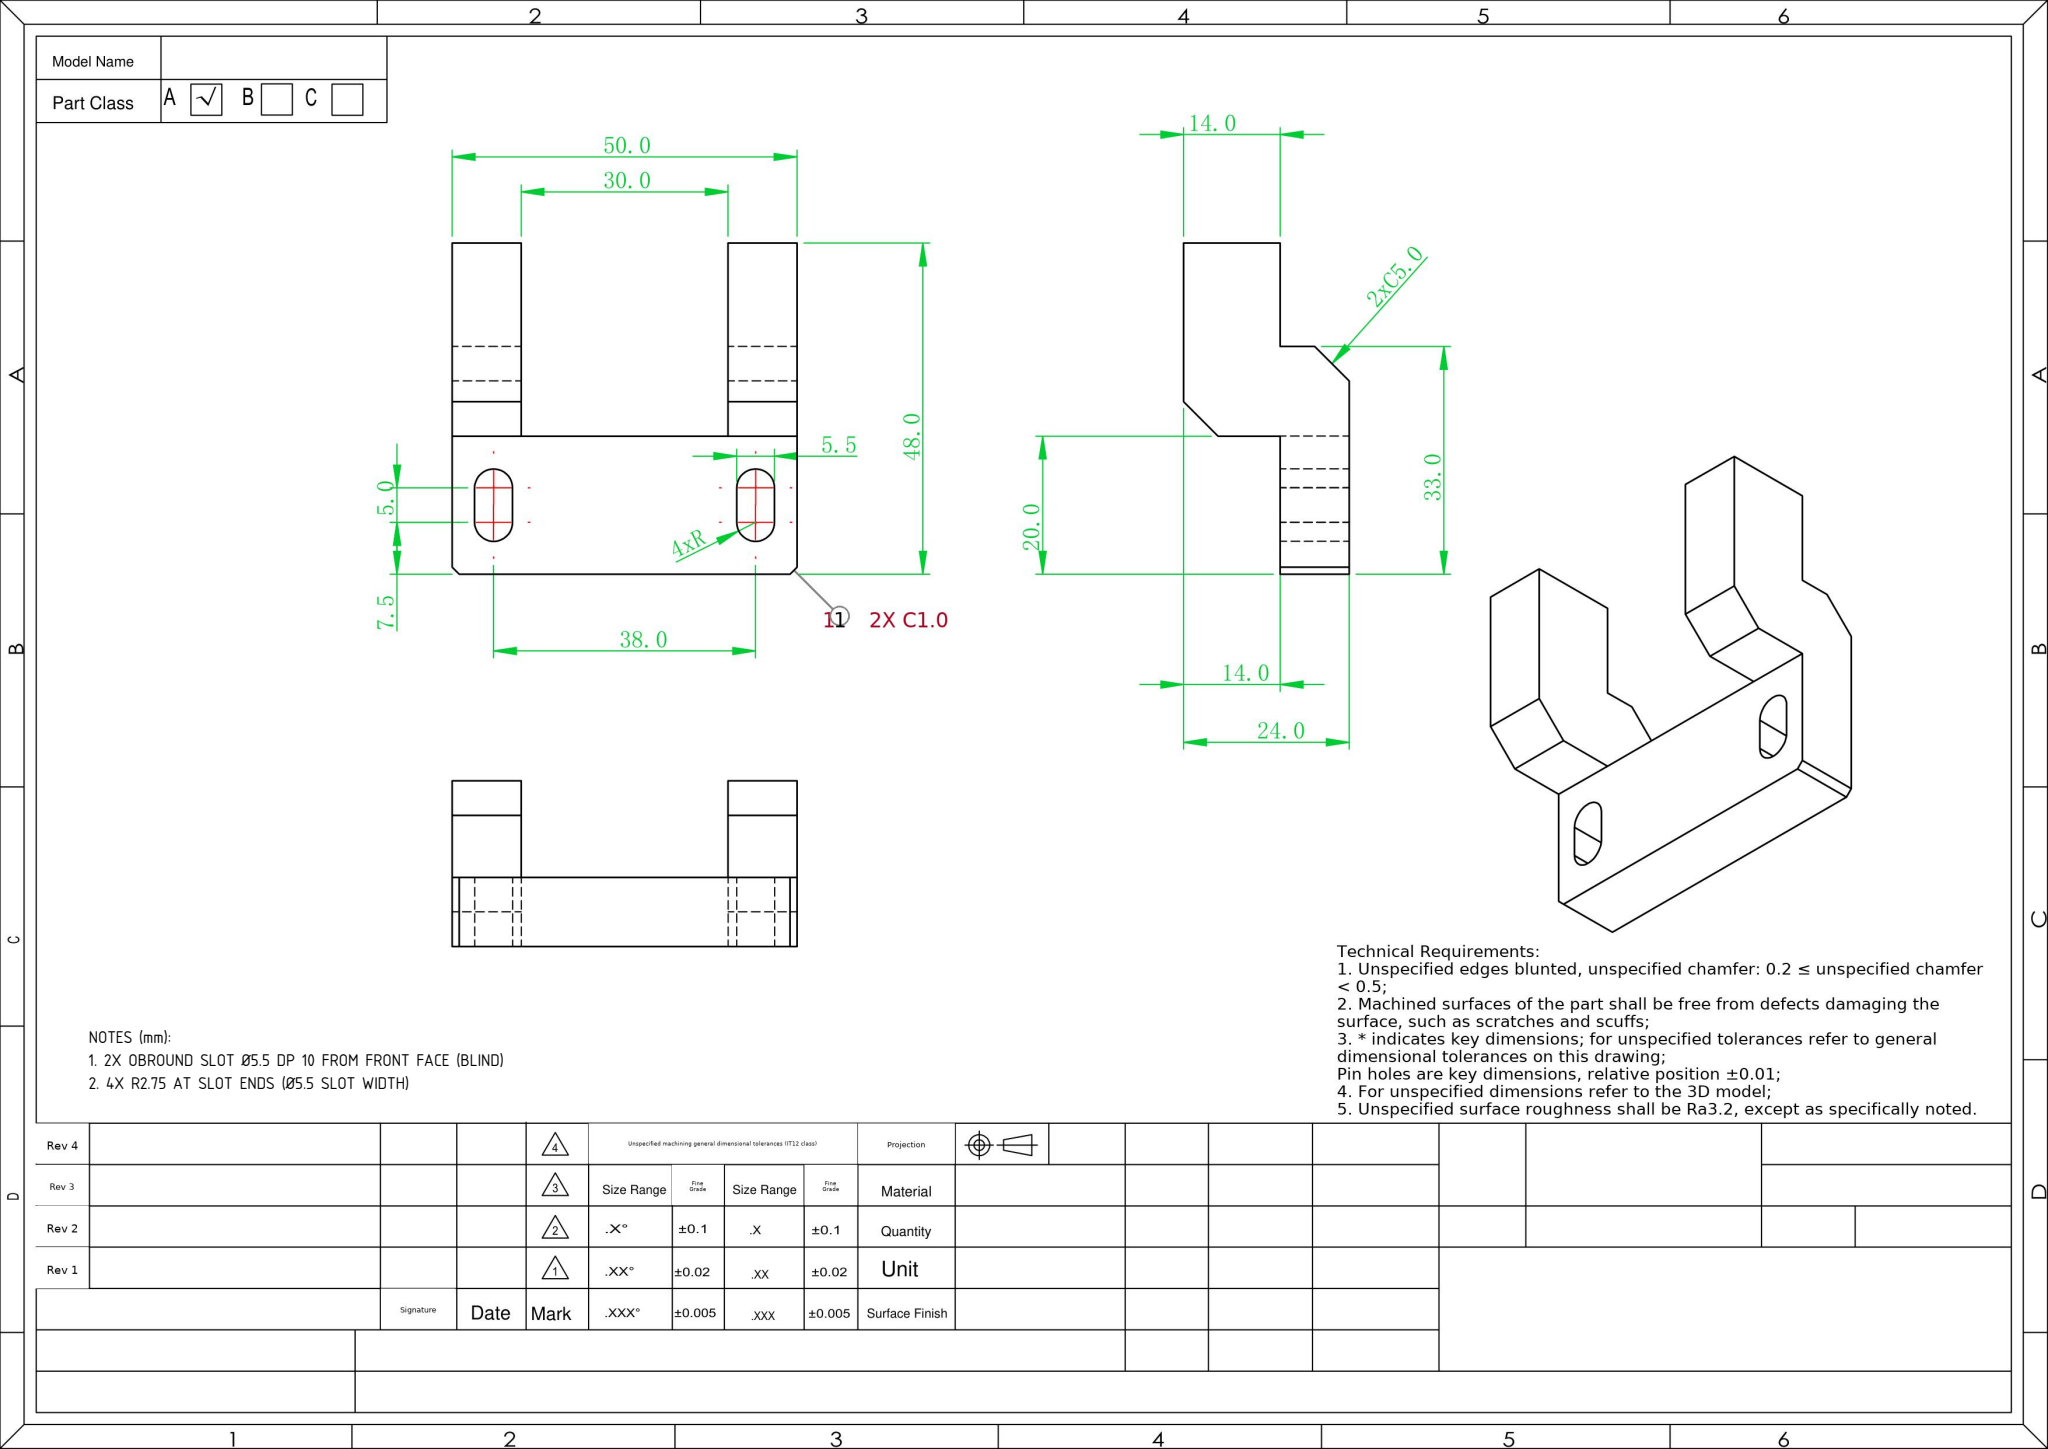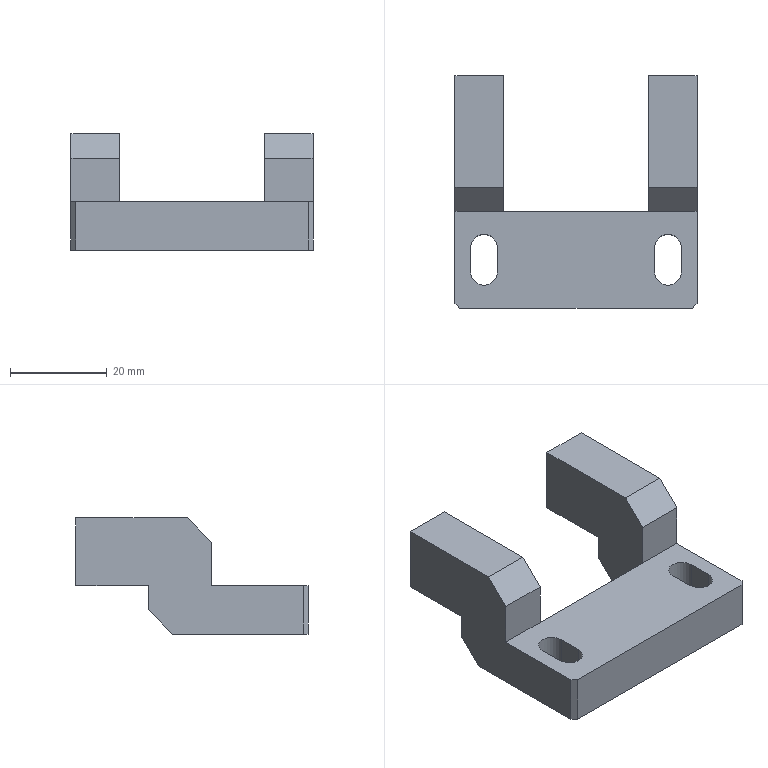Part | SolidWorks | mm | 1 solid | 32 faces | box 50 x 48 x 24 mm | volume 18905 mm3 | plane 28 | cylinder 4 | commonest cylinder face diameters 5.5 x4
Drawing notes:
2X OBROUND SLOT Ø5.5 DP 10 FROM FRONT FACE (BLIND) | from the solid: 4 cylinders Ø5.5, axis z, length 10.0, starting at z=0 (part z-extent 24.0)
4X R2.75 AT SLOT ENDS (Ø5.5 SLOT WIDTH) | from the solid: 4 cylinders dia 5.5 axis z at (6,7.5),(6,12.5),(44,7.5),(44,12.5) -> R2.75 ends
build123d program:
from build123d import *

# Parameters (mm, degrees)
SKETCH1_W           = 50
SKETCH1_H           = 48
BOSS_EXTRUDE1_DEPTH = 24
SKETCH2_W           = 30
SKETCH2_H           = 56
CUT_EXTRUDE1_DEPTH  = 43.154
SKETCH3_W           = 10
SKETCH3_H           = 15
CUT_EXTRUDE2_DEPTH  = 61.432
SKETCH4_W           = 30
SKETCH4_H           = 40
CUT_EXTRUDE4_DEPTH  = 14
SKETCH5_W           = 14
SKETCH5_H           = 20
CUT_EXTRUDE5_DEPTH  = 61.432
CHAMFER2_SIZE       = 5
CUT_EXTRUDE6_DEPTH  = 38.376
CHAMFER3_SIZE       = 1


with BuildPart() as part:
    # Sketch1 → Boss-Extrude1 (new body)
    with BuildSketch(Plane.XY):
        Rectangle(SKETCH1_W, SKETCH1_H)
    extrude(amount=BOSS_EXTRUDE1_DEPTH)

    # Sketch2 → Cut-Extrude1 (cut, through all)
    with BuildSketch(Plane.XY.offset(24)):
        with Locations((0, 24)):
            Rectangle(SKETCH2_W, SKETCH2_H)
    extrude(amount=-CUT_EXTRUDE1_DEPTH, mode=Mode.SUBTRACT)

    # Sketch3 → Cut-Extrude2 (cut, through all)
    with BuildSketch(Plane.ZY.offset(25)):
        with Locations((5, 16.5)):
            Rectangle(SKETCH3_W, SKETCH3_H)
    extrude(amount=-CUT_EXTRUDE2_DEPTH, mode=Mode.SUBTRACT)

    # Sketch4 → Cut-Extrude4 (cut)
    with BuildSketch(Plane.XY.offset(24)):
        with Locations((0, -4)):
            Rectangle(SKETCH4_W, SKETCH4_H)
    extrude(amount=-CUT_EXTRUDE4_DEPTH, mode=Mode.SUBTRACT)

    # Sketch5 → Cut-Extrude5 (cut, through all)
    with BuildSketch(Plane.ZY.offset(25)):
        with Locations((17, -14)):
            Rectangle(SKETCH5_W, SKETCH5_H)
    extrude(amount=-CUT_EXTRUDE5_DEPTH, mode=Mode.SUBTRACT)

    # Chamfer2
    chamfer2_edges = [part.edges().sort_by_distance(p)[0] for p in [
        (20, 9, 0),
        (-20, 9, 0),
        (20, -4, 24),
        (-20, -4, 24),
    ]]
    chamfer(chamfer2_edges, length=CHAMFER2_SIZE)

    # Sketch6 → Cut-Extrude6 (cut, through all)
    with BuildSketch(Plane.XY.offset(10)):
        with BuildLine():
            Line((-16.25, -11.5), (-16.25, -16.5))
            ThreePointArc((-16.25, -16.5), (-19, -19.25), (-21.75, -16.5))
            Line((-21.75, -16.5), (-21.75, -11.5))
            ThreePointArc((-21.75, -11.5), (-19, -8.75), (-16.25, -11.5))
        make_face()
        with BuildLine():
            Line((21.75, -11.5), (21.75, -16.5))
            ThreePointArc((21.75, -16.5), (19, -19.25), (16.25, -16.5))
            Line((16.25, -16.5), (16.25, -11.5))
            ThreePointArc((16.25, -11.5), (19, -8.75), (21.75, -11.5))
        make_face()
    extrude(amount=-CUT_EXTRUDE6_DEPTH, mode=Mode.SUBTRACT)

    # Chamfer3
    chamfer3_edges = [part.edges().sort_by_distance(p)[0] for p in [
        (25, -24, 5),
        (-25, -24, 5),
    ]]
    chamfer(chamfer3_edges, length=CHAMFER3_SIZE)


solid = part.part
STEP:
#1=CARTESIAN_POINT('',(15.,1.,24.));
#2=VERTEX_POINT('',#1);
#3=CARTESIAN_POINT('',(15.,24.,24.));
#4=VERTEX_POINT('',#3);
#5=CARTESIAN_POINT('',(15.,52.,24.));
#6=DIRECTION('',(-0.,1.,0.));
#7=VECTOR('',#6,1000.);
#8=LINE('',#5,#7);
#9=EDGE_CURVE('',#2,#4,#8,.T.);
#10=ORIENTED_EDGE('',*,*,#9,.F.);
#11=CARTESIAN_POINT('',(25.,1.,24.));
#12=VERTEX_POINT('',#11);
#13=CARTESIAN_POINT('',(25.,1.,24.));
#14=DIRECTION('',(1.,0.,0.));
#15=VECTOR('',#14,1000.);
#16=LINE('',#13,#15);
#17=EDGE_CURVE('',#2,#12,#16,.T.);
#18=ORIENTED_EDGE('',*,*,#17,.T.);
#19=CARTESIAN_POINT('',(25.,24.,24.));
#20=VERTEX_POINT('',#19);
#21=CARTESIAN_POINT('',(25.,-24.,24.));
#22=DIRECTION('',(0.,1.,0.));
#23=VECTOR('',#22,1000.);
#24=LINE('',#21,#23);
#25=EDGE_CURVE('',#12,#20,#24,.T.);
#26=ORIENTED_EDGE('',*,*,#25,.T.);
#27=CARTESIAN_POINT('',(25.,24.,24.));
#28=DIRECTION('',(-1.,-0.,0.));
#29=VECTOR('',#28,1000.);
#30=LINE('',#27,#29);
#31=EDGE_CURVE('',#20,#4,#30,.T.);
#32=ORIENTED_EDGE('',*,*,#31,.T.);
#33=EDGE_LOOP('',(#10,#18,#26,#32));
#34=FACE_OUTER_BOUND('',#33,.T.);
#35=CARTESIAN_POINT('',(0.,0.,24.));
#36=DIRECTION('',(0.,0.,1.));
#37=DIRECTION('',(1.,0.,0.));
#38=AXIS2_PLACEMENT_3D('',#35,#36,#37);
#39=PLANE('',#38);
#40=ADVANCED_FACE('',(#34),#39,.T.);
#41=CARTESIAN_POINT('',(15.,-4.,10.));
#42=VERTEX_POINT('',#41);
#43=CARTESIAN_POINT('',(-15.,-4.,10.));
#44=VERTEX_POINT('',#43);
#45=CARTESIAN_POINT('',(-15.,-4.,10.));
#46=DIRECTION('',(-1.,0.,0.));
#47=VECTOR('',#46,1000.);
#48=LINE('',#45,#47);
#49=EDGE_CURVE('',#42,#44,#48,.T.);
#50=ORIENTED_EDGE('',*,*,#49,.F.);
#51=CARTESIAN_POINT('',(15.,-4.,0.));
#52=VERTEX_POINT('',#51);
#53=CARTESIAN_POINT('',(15.,-4.,0.));
#54=DIRECTION('',(0.,0.,1.));
#55=VECTOR('',#54,1000.);
#56=LINE('',#53,#55);
#57=EDGE_CURVE('',#52,#42,#56,.T.);
#58=ORIENTED_EDGE('',*,*,#57,.F.);
#59=CARTESIAN_POINT('',(-15.,-4.,0.));
#60=VERTEX_POINT('',#59);
#61=CARTESIAN_POINT('',(-15.,-4.,0.));
#62=DIRECTION('',(1.,0.,0.));
#63=VECTOR('',#62,1000.);
#64=LINE('',#61,#63);
#65=EDGE_CURVE('',#60,#52,#64,.T.);
#66=ORIENTED_EDGE('',*,*,#65,.F.);
#67=CARTESIAN_POINT('',(-15.,-4.,0.));
#68=DIRECTION('',(0.,0.,1.));
#69=VECTOR('',#68,1000.);
#70=LINE('',#67,#69);
#71=EDGE_CURVE('',#60,#44,#70,.T.);
#72=ORIENTED_EDGE('',*,*,#71,.T.);
#73=EDGE_LOOP('',(#50,#58,#66,#72));
#74=FACE_OUTER_BOUND('',#73,.T.);
#75=CARTESIAN_POINT('',(-15.,-4.,0.));
#76=DIRECTION('',(0.,-1.,0.));
#77=DIRECTION('',(0.,0.,-1.));
#78=AXIS2_PLACEMENT_3D('',#75,#76,#77);
#79=PLANE('',#78);
#80=ADVANCED_FACE('',(#74),#79,.F.);
#81=CARTESIAN_POINT('',(25.,24.,10.));
#82=VERTEX_POINT('',#81);
#83=CARTESIAN_POINT('',(25.,24.,24.));
#84=DIRECTION('',(0.,0.,-1.));
#85=VECTOR('',#84,1000.);
#86=LINE('',#83,#85);
#87=EDGE_CURVE('',#20,#82,#86,.T.);
#88=ORIENTED_EDGE('',*,*,#87,.T.);
#89=CARTESIAN_POINT('',(15.,24.,10.));
#90=VERTEX_POINT('',#89);
#91=CARTESIAN_POINT('',(25.,24.,10.));
#92=DIRECTION('',(-1.,0.,0.));
#93=VECTOR('',#92,1000.);
#94=LINE('',#91,#93);
#95=EDGE_CURVE('',#82,#90,#94,.T.);
#96=ORIENTED_EDGE('',*,*,#95,.T.);
#97=CARTESIAN_POINT('',(15.,24.,24.));
#98=DIRECTION('',(0.,0.,1.));
#99=VECTOR('',#98,1000.);
#100=LINE('',#97,#99);
#101=EDGE_CURVE('',#90,#4,#100,.T.);
#102=ORIENTED_EDGE('',*,*,#101,.T.);
#103=ORIENTED_EDGE('',*,*,#31,.F.);
#104=EDGE_LOOP('',(#88,#96,#102,#103));
#105=FACE_OUTER_BOUND('',#104,.T.);
#106=CARTESIAN_POINT('',(25.,24.,24.));
#107=DIRECTION('',(0.,-1.,0.));
#108=DIRECTION('',(1.,0.,0.));
#109=AXIS2_PLACEMENT_3D('',#106,#107,#108);
#110=PLANE('',#109);
#111=ADVANCED_FACE('',(#105),#110,.F.);
#112=CARTESIAN_POINT('',(-25.,4.,0.));
#113=VERTEX_POINT('',#112);
#114=CARTESIAN_POINT('',(-25.,-23.,0.));
#115=VERTEX_POINT('',#114);
#116=CARTESIAN_POINT('',(-25.,-24.,0.));
#117=DIRECTION('',(0.,-1.,0.));
#118=VECTOR('',#117,1000.);
#119=LINE('',#116,#118);
#120=EDGE_CURVE('',#113,#115,#119,.T.);
#121=ORIENTED_EDGE('',*,*,#120,.T.);
#122=CARTESIAN_POINT('',(-25.,-23.,10.));
#123=VERTEX_POINT('',#122);
#124=CARTESIAN_POINT('',(-25.,-23.,24.));
#125=DIRECTION('',(0.,0.,1.));
#126=VECTOR('',#125,1000.);
#127=LINE('',#124,#126);
#128=EDGE_CURVE('',#115,#123,#127,.T.);
#129=ORIENTED_EDGE('',*,*,#128,.T.);
#130=CARTESIAN_POINT('',(-25.,-4.,10.));
#131=VERTEX_POINT('',#130);
#132=CARTESIAN_POINT('',(-25.,-24.,10.));
#133=DIRECTION('',(0.,-1.,0.));
#134=VECTOR('',#133,1000.);
#135=LINE('',#132,#134);
#136=EDGE_CURVE('',#131,#123,#135,.T.);
#137=ORIENTED_EDGE('',*,*,#136,.F.);
#138=CARTESIAN_POINT('',(-25.,-4.,19.));
#139=VERTEX_POINT('',#138);
#140=CARTESIAN_POINT('',(-25.,-4.,24.));
#141=DIRECTION('',(0.,0.,-1.));
#142=VECTOR('',#141,1000.);
#143=LINE('',#140,#142);
#144=EDGE_CURVE('',#139,#131,#143,.T.);
#145=ORIENTED_EDGE('',*,*,#144,.F.);
#146=CARTESIAN_POINT('',(-25.,1.,24.));
#147=VERTEX_POINT('',#146);
#148=CARTESIAN_POINT('',(-25.,-4.,19.));
#149=DIRECTION('',(0.,0.7071,0.7071));
#150=VECTOR('',#149,1000.);
#151=LINE('',#148,#150);
#152=EDGE_CURVE('',#139,#147,#151,.T.);
#153=ORIENTED_EDGE('',*,*,#152,.T.);
#154=CARTESIAN_POINT('',(-25.,24.,24.));
#155=VERTEX_POINT('',#154);
#156=CARTESIAN_POINT('',(-25.,-24.,24.));
#157=DIRECTION('',(0.,-1.,0.));
#158=VECTOR('',#157,1000.);
#159=LINE('',#156,#158);
#160=EDGE_CURVE('',#155,#147,#159,.T.);
#161=ORIENTED_EDGE('',*,*,#160,.F.);
#162=CARTESIAN_POINT('',(-25.,24.,10.));
#163=VERTEX_POINT('',#162);
#164=CARTESIAN_POINT('',(-25.,24.,24.));
#165=DIRECTION('',(0.,0.,-1.));
#166=VECTOR('',#165,1000.);
#167=LINE('',#164,#166);
#168=EDGE_CURVE('',#155,#163,#167,.T.);
#169=ORIENTED_EDGE('',*,*,#168,.T.);
#170=CARTESIAN_POINT('',(-25.,9.,10.));
#171=VERTEX_POINT('',#170);
#172=CARTESIAN_POINT('',(-25.,24.,10.));
#173=DIRECTION('',(0.,1.,0.));
#174=VECTOR('',#173,1000.);
#175=LINE('',#172,#174);
#176=EDGE_CURVE('',#171,#163,#175,.T.);
#177=ORIENTED_EDGE('',*,*,#176,.F.);
#178=CARTESIAN_POINT('',(-25.,9.,5.));
#179=VERTEX_POINT('',#178);
#180=CARTESIAN_POINT('',(-25.,9.,0.));
#181=DIRECTION('',(0.,0.,1.));
#182=VECTOR('',#181,1000.);
#183=LINE('',#180,#182);
#184=EDGE_CURVE('',#179,#171,#183,.T.);
#185=ORIENTED_EDGE('',*,*,#184,.F.);
#186=CARTESIAN_POINT('',(-25.,9.,5.));
#187=DIRECTION('',(0.,-0.7071,-0.7071));
#188=VECTOR('',#187,1000.);
#189=LINE('',#186,#188);
#190=EDGE_CURVE('',#179,#113,#189,.T.);
#191=ORIENTED_EDGE('',*,*,#190,.T.);
#192=EDGE_LOOP('',(#121,#129,#137,#145,#153,#161,#169,#177,#185,#191));
#193=FACE_OUTER_BOUND('',#192,.T.);
#194=CARTESIAN_POINT('',(-25.,-24.,24.));
#195=DIRECTION('',(1.,0.,0.));
#196=DIRECTION('',(0.,0.,-1.));
#197=AXIS2_PLACEMENT_3D('',#194,#195,#196);
#198=PLANE('',#197);
#199=ADVANCED_FACE('',(#193),#198,.F.);
#200=CARTESIAN_POINT('',(-24.,-24.,0.));
#201=VERTEX_POINT('',#200);
#202=CARTESIAN_POINT('',(24.,-24.,0.));
#203=VERTEX_POINT('',#202);
#204=CARTESIAN_POINT('',(25.,-24.,0.));
#205=DIRECTION('',(1.,0.,0.));
#206=VECTOR('',#205,1000.);
#207=LINE('',#204,#206);
#208=EDGE_CURVE('',#201,#203,#207,.T.);
#209=ORIENTED_EDGE('',*,*,#208,.T.);
#210=CARTESIAN_POINT('',(24.,-24.,10.));
#211=VERTEX_POINT('',#210);
#212=CARTESIAN_POINT('',(24.,-24.,24.));
#213=DIRECTION('',(0.,0.,1.));
#214=VECTOR('',#213,1000.);
#215=LINE('',#212,#214);
#216=EDGE_CURVE('',#203,#211,#215,.T.);
#217=ORIENTED_EDGE('',*,*,#216,.T.);
#218=CARTESIAN_POINT('',(-24.,-24.,10.));
#219=VERTEX_POINT('',#218);
#220=CARTESIAN_POINT('',(-15.,-24.,10.));
#221=DIRECTION('',(1.,0.,0.));
#222=VECTOR('',#221,1000.);
#223=LINE('',#220,#222);
#224=EDGE_CURVE('',#219,#211,#223,.T.);
#225=ORIENTED_EDGE('',*,*,#224,.F.);
#226=CARTESIAN_POINT('',(-24.,-24.,24.));
#227=DIRECTION('',(0.,0.,-1.));
#228=VECTOR('',#227,1000.);
#229=LINE('',#226,#228);
#230=EDGE_CURVE('',#219,#201,#229,.T.);
#231=ORIENTED_EDGE('',*,*,#230,.T.);
#232=EDGE_LOOP('',(#209,#217,#225,#231));
#233=FACE_OUTER_BOUND('',#232,.T.);
#234=CARTESIAN_POINT('',(25.,-24.,24.));
#235=DIRECTION('',(-0.,1.,0.));
#236=DIRECTION('',(-1.,-0.,0.));
#237=AXIS2_PLACEMENT_3D('',#234,#235,#236);
#238=PLANE('',#237);
#239=ADVANCED_FACE('',(#233),#238,.F.);
#240=CARTESIAN_POINT('',(25.,-4.,10.));
#241=VERTEX_POINT('',#240);
#242=CARTESIAN_POINT('',(25.,-23.,10.));
#243=VERTEX_POINT('',#242);
#244=CARTESIAN_POINT('',(25.,-24.,10.));
#245=DIRECTION('',(0.,-1.,0.));
#246=VECTOR('',#245,1000.);
#247=LINE('',#244,#246);
#248=EDGE_CURVE('',#241,#243,#247,.T.);
#249=ORIENTED_EDGE('',*,*,#248,.T.);
#250=CARTESIAN_POINT('',(25.,-23.,0.));
#251=VERTEX_POINT('',#250);
#252=CARTESIAN_POINT('',(25.,-23.,24.));
#253=DIRECTION('',(0.,0.,-1.));
#254=VECTOR('',#253,1000.);
#255=LINE('',#252,#254);
#256=EDGE_CURVE('',#243,#251,#255,.T.);
#257=ORIENTED_EDGE('',*,*,#256,.T.);
#258=CARTESIAN_POINT('',(25.,4.,0.));
#259=VERTEX_POINT('',#258);
#260=CARTESIAN_POINT('',(25.,-24.,0.));
#261=DIRECTION('',(0.,1.,0.));
#262=VECTOR('',#261,1000.);
#263=LINE('',#260,#262);
#264=EDGE_CURVE('',#251,#259,#263,.T.);
#265=ORIENTED_EDGE('',*,*,#264,.T.);
#266=CARTESIAN_POINT('',(25.,9.,5.));
#267=VERTEX_POINT('',#266);
#268=CARTESIAN_POINT('',(25.,9.,5.));
#269=DIRECTION('',(0.,0.7071,0.7071));
#270=VECTOR('',#269,1000.);
#271=LINE('',#268,#270);
#272=EDGE_CURVE('',#259,#267,#271,.T.);
#273=ORIENTED_EDGE('',*,*,#272,.T.);
#274=CARTESIAN_POINT('',(25.,9.,10.));
#275=VERTEX_POINT('',#274);
#276=CARTESIAN_POINT('',(25.,9.,0.));
#277=DIRECTION('',(0.,0.,1.));
#278=VECTOR('',#277,1000.);
#279=LINE('',#276,#278);
#280=EDGE_CURVE('',#267,#275,#279,.T.);
#281=ORIENTED_EDGE('',*,*,#280,.T.);
#282=CARTESIAN_POINT('',(25.,24.,10.));
#283=DIRECTION('',(0.,1.,0.));
#284=VECTOR('',#283,1000.);
#285=LINE('',#282,#284);
#286=EDGE_CURVE('',#275,#82,#285,.T.);
#287=ORIENTED_EDGE('',*,*,#286,.T.);
#288=ORIENTED_EDGE('',*,*,#87,.F.);
#289=ORIENTED_EDGE('',*,*,#25,.F.);
#290=CARTESIAN_POINT('',(25.,-4.,19.));
#291=VERTEX_POINT('',#290);
#292=CARTESIAN_POINT('',(25.,-4.,19.));
#293=DIRECTION('',(0.,-0.7071,-0.7071));
#294=VECTOR('',#293,1000.);
#295=LINE('',#292,#294);
#296=EDGE_CURVE('',#12,#291,#295,.T.);
#297=ORIENTED_EDGE('',*,*,#296,.T.);
#298=CARTESIAN_POINT('',(25.,-4.,24.));
#299=DIRECTION('',(0.,0.,-1.));
#300=VECTOR('',#299,1000.);
#301=LINE('',#298,#300);
#302=EDGE_CURVE('',#291,#241,#301,.T.);
#303=ORIENTED_EDGE('',*,*,#302,.T.);
#304=EDGE_LOOP('',(#249,#257,#265,#273,#281,#287,#288,#289,#297,#303));
#305=FACE_OUTER_BOUND('',#304,.T.);
#306=CARTESIAN_POINT('',(25.,-24.,24.));
#307=DIRECTION('',(-1.,0.,0.));
#308=DIRECTION('',(0.,0.,1.));
#309=AXIS2_PLACEMENT_3D('',#306,#307,#308);
#310=PLANE('',#309);
#311=ADVANCED_FACE('',(#305),#310,.F.);
#312=CARTESIAN_POINT('',(-15.,24.,24.));
#313=VERTEX_POINT('',#312);
#314=CARTESIAN_POINT('',(-15.,24.,10.));
#315=VERTEX_POINT('',#314);
#316=CARTESIAN_POINT('',(-15.,24.,24.));
#317=DIRECTION('',(0.,0.,-1.));
#318=VECTOR('',#317,1000.);
#319=LINE('',#316,#318);
#320=EDGE_CURVE('',#313,#315,#319,.T.);
#321=ORIENTED_EDGE('',*,*,#320,.T.);
#322=CARTESIAN_POINT('',(25.,24.,10.));
#323=DIRECTION('',(-1.,0.,0.));
#324=VECTOR('',#323,1000.);
#325=LINE('',#322,#324);
#326=EDGE_CURVE('',#315,#163,#325,.T.);
#327=ORIENTED_EDGE('',*,*,#326,.T.);
#328=ORIENTED_EDGE('',*,*,#168,.F.);
#329=CARTESIAN_POINT('',(25.,24.,24.));
#330=DIRECTION('',(-1.,-0.,0.));
#331=VECTOR('',#330,1000.);
#332=LINE('',#329,#331);
#333=EDGE_CURVE('',#313,#155,#332,.T.);
#334=ORIENTED_EDGE('',*,*,#333,.F.);
#335=EDGE_LOOP('',(#321,#327,#328,#334));
#336=FACE_OUTER_BOUND('',#335,.T.);
#337=CARTESIAN_POINT('',(25.,24.,24.));
#338=DIRECTION('',(0.,-1.,0.));
#339=DIRECTION('',(1.,0.,0.));
#340=AXIS2_PLACEMENT_3D('',#337,#338,#339);
#341=PLANE('',#340);
#342=ADVANCED_FACE('',(#336),#341,.F.);
#343=ORIENTED_EDGE('',*,*,#160,.T.);
#344=CARTESIAN_POINT('',(-15.,1.,24.));
#345=VERTEX_POINT('',#344);
#346=CARTESIAN_POINT('',(-15.,1.,24.));
#347=DIRECTION('',(1.,0.,0.));
#348=VECTOR('',#347,1000.);
#349=LINE('',#346,#348);
#350=EDGE_CURVE('',#147,#345,#349,.T.);
#351=ORIENTED_EDGE('',*,*,#350,.T.);
#352=CARTESIAN_POINT('',(-15.,52.,24.));
#353=DIRECTION('',(0.,-1.,0.));
#354=VECTOR('',#353,1000.);
#355=LINE('',#352,#354);
#356=EDGE_CURVE('',#313,#345,#355,.T.);
#357=ORIENTED_EDGE('',*,*,#356,.F.);
#358=ORIENTED_EDGE('',*,*,#333,.T.);
#359=EDGE_LOOP('',(#343,#351,#357,#358));
#360=FACE_OUTER_BOUND('',#359,.T.);
#361=CARTESIAN_POINT('',(0.,0.,24.));
#362=DIRECTION('',(0.,0.,1.));
#363=DIRECTION('',(1.,0.,0.));
#364=AXIS2_PLACEMENT_3D('',#361,#362,#363);
#365=PLANE('',#364);
#366=ADVANCED_FACE('',(#360),#365,.T.);
#367=CARTESIAN_POINT('',(-16.25,-16.5,0.));
#368=VERTEX_POINT('',#367);
#369=CARTESIAN_POINT('',(-16.25,-11.5,0.));
#370=VERTEX_POINT('',#369);
#371=CARTESIAN_POINT('',(-16.25,-11.5,0.));
#372=DIRECTION('',(0.,1.,0.));
#373=VECTOR('',#372,1000.);
#374=LINE('',#371,#373);
#375=EDGE_CURVE('',#368,#370,#374,.T.);
#376=ORIENTED_EDGE('',*,*,#375,.T.);
#377=CARTESIAN_POINT('',(-21.75,-11.5,0.));
#378=VERTEX_POINT('',#377);
#379=CARTESIAN_POINT('',(-19.,-11.5,0.));
#380=DIRECTION('',(0.,0.,1.));
#381=DIRECTION('',(1.,0.,0.));
#382=AXIS2_PLACEMENT_3D('',#379,#380,#381);
#383=CIRCLE('',#382,2.75);
#384=EDGE_CURVE('',#370,#378,#383,.T.);
#385=ORIENTED_EDGE('',*,*,#384,.T.);
#386=CARTESIAN_POINT('',(-21.75,-16.5,0.));
#387=VERTEX_POINT('',#386);
#388=CARTESIAN_POINT('',(-21.75,-11.5,0.));
#389=DIRECTION('',(0.,-1.,0.));
#390=VECTOR('',#389,1000.);
#391=LINE('',#388,#390);
#392=EDGE_CURVE('',#378,#387,#391,.T.);
#393=ORIENTED_EDGE('',*,*,#392,.T.);
#394=CARTESIAN_POINT('',(-19.,-16.5,0.));
#395=DIRECTION('',(0.,0.,1.));
#396=DIRECTION('',(1.,0.,0.));
#397=AXIS2_PLACEMENT_3D('',#394,#395,#396);
#398=CIRCLE('',#397,2.75);
#399=EDGE_CURVE('',#387,#368,#398,.T.);
#400=ORIENTED_EDGE('',*,*,#399,.T.);
#401=EDGE_LOOP('',(#376,#385,#393,#400));
#402=FACE_BOUND('',#401,.T.);
#403=CARTESIAN_POINT('',(21.75,-16.5,0.));
#404=VERTEX_POINT('',#403);
#405=CARTESIAN_POINT('',(21.75,-11.5,0.));
#406=VERTEX_POINT('',#405);
#407=CARTESIAN_POINT('',(21.75,-11.5,0.));
#408=DIRECTION('',(0.,1.,0.));
#409=VECTOR('',#408,1000.);
#410=LINE('',#407,#409);
#411=EDGE_CURVE('',#404,#406,#410,.T.);
#412=ORIENTED_EDGE('',*,*,#411,.T.);
#413=CARTESIAN_POINT('',(16.25,-11.5,0.));
#414=VERTEX_POINT('',#413);
#415=CARTESIAN_POINT('',(19.,-11.5,0.));
#416=DIRECTION('',(0.,0.,1.));
#417=DIRECTION('',(1.,0.,0.));
#418=AXIS2_PLACEMENT_3D('',#415,#416,#417);
#419=CIRCLE('',#418,2.75);
#420=EDGE_CURVE('',#406,#414,#419,.T.);
#421=ORIENTED_EDGE('',*,*,#420,.T.);
#422=CARTESIAN_POINT('',(16.25,-16.5,0.));
#423=VERTEX_POINT('',#422);
#424=CARTESIAN_POINT('',(16.25,-11.5,0.));
#425=DIRECTION('',(0.,-1.,0.));
#426=VECTOR('',#425,1000.);
#427=LINE('',#424,#426);
#428=EDGE_CURVE('',#414,#423,#427,.T.);
#429=ORIENTED_EDGE('',*,*,#428,.T.);
#430=CARTESIAN_POINT('',(19.,-16.5,0.));
#431=DIRECTION('',(0.,0.,1.));
#432=DIRECTION('',(1.,0.,0.));
#433=AXIS2_PLACEMENT_3D('',#430,#431,#432);
#434=CIRCLE('',#433,2.75);
#435=EDGE_CURVE('',#423,#404,#434,.T.);
#436=ORIENTED_EDGE('',*,*,#435,.T.);
#437=EDGE_LOOP('',(#412,#421,#429,#436));
#438=FACE_BOUND('',#437,.T.);
#439=ORIENTED_EDGE('',*,*,#264,.F.);
#440=CARTESIAN_POINT('',(25.,-23.,0.));
#441=DIRECTION('',(-0.7071,-0.7071,0.));
#442=VECTOR('',#441,1000.);
#443=LINE('',#440,#442);
#444=EDGE_CURVE('',#251,#203,#443,.T.);
#445=ORIENTED_EDGE('',*,*,#444,.T.);
#446=ORIENTED_EDGE('',*,*,#208,.F.);
#447=CARTESIAN_POINT('',(-24.,-24.,0.));
#448=DIRECTION('',(-0.7071,0.7071,0.));
#449=VECTOR('',#448,1000.);
#450=LINE('',#447,#449);
#451=EDGE_CURVE('',#201,#115,#450,.T.);
#452=ORIENTED_EDGE('',*,*,#451,.T.);
#453=ORIENTED_EDGE('',*,*,#120,.F.);
#454=CARTESIAN_POINT('',(-15.,4.,0.));
#455=VERTEX_POINT('',#454);
#456=CARTESIAN_POINT('',(0.,4.,0.));
#457=DIRECTION('',(1.,0.,0.));
#458=VECTOR('',#457,1000.);
#459=LINE('',#456,#458);
#460=EDGE_CURVE('',#113,#455,#459,.T.);
#461=ORIENTED_EDGE('',*,*,#460,.T.);
#462=CARTESIAN_POINT('',(-15.,-0.,0.));
#463=DIRECTION('',(0.,-1.,0.));
#464=VECTOR('',#463,1000.);
#465=LINE('',#462,#464);
#466=EDGE_CURVE('',#455,#60,#465,.T.);
#467=ORIENTED_EDGE('',*,*,#466,.T.);
#468=ORIENTED_EDGE('',*,*,#65,.T.);
#469=CARTESIAN_POINT('',(15.,4.,0.));
#470=VERTEX_POINT('',#469);
#471=CARTESIAN_POINT('',(15.,52.,0.));
#472=DIRECTION('',(-0.,1.,0.));
#473=VECTOR('',#472,1000.);
#474=LINE('',#471,#473);
#475=EDGE_CURVE('',#52,#470,#474,.T.);
#476=ORIENTED_EDGE('',*,*,#475,.T.);
#477=CARTESIAN_POINT('',(0.,4.,0.));
#478=DIRECTION('',(1.,0.,0.));
#479=VECTOR('',#478,1000.);
#480=LINE('',#477,#479);
#481=EDGE_CURVE('',#470,#259,#480,.T.);
#482=ORIENTED_EDGE('',*,*,#481,.T.);
#483=EDGE_LOOP('',(#439,#445,#446,#452,#453,#461,#467,#468,#476,#482));
#484=FACE_OUTER_BOUND('',#483,.T.);
#485=CARTESIAN_POINT('',(0.,0.,0.));
#486=DIRECTION('',(0.,0.,1.));
#487=DIRECTION('',(1.,0.,0.));
#488=AXIS2_PLACEMENT_3D('',#485,#486,#487);
#489=PLANE('',#488);
#490=ADVANCED_FACE('',(#402,#438,#484),#489,.F.);
#491=CARTESIAN_POINT('',(15.,-4.,19.));
#492=VERTEX_POINT('',#491);
#493=CARTESIAN_POINT('',(15.,-4.,0.));
#494=DIRECTION('',(0.,0.,1.));
#495=VECTOR('',#494,1000.);
#496=LINE('',#493,#495);
#497=EDGE_CURVE('',#42,#492,#496,.T.);
#498=ORIENTED_EDGE('',*,*,#497,.T.);
#499=CARTESIAN_POINT('',(15.,-4.,19.));
#500=DIRECTION('',(-0.,0.7071,0.7071));
#501=VECTOR('',#500,1000.);
#502=LINE('',#499,#501);
#503=EDGE_CURVE('',#492,#2,#502,.T.);
#504=ORIENTED_EDGE('',*,*,#503,.T.);
#505=ORIENTED_EDGE('',*,*,#9,.T.);
#506=ORIENTED_EDGE('',*,*,#101,.F.);
#507=CARTESIAN_POINT('',(15.,9.,10.));
#508=VERTEX_POINT('',#507);
#509=CARTESIAN_POINT('',(15.,52.,10.));
#510=DIRECTION('',(0.,-1.,0.));
#511=VECTOR('',#510,1000.);
#512=LINE('',#509,#511);
#513=EDGE_CURVE('',#90,#508,#512,.T.);
#514=ORIENTED_EDGE('',*,*,#513,.T.);
#515=CARTESIAN_POINT('',(15.,9.,5.));
#516=VERTEX_POINT('',#515);
#517=CARTESIAN_POINT('',(15.,9.,0.));
#518=DIRECTION('',(0.,0.,-1.));
#519=VECTOR('',#518,1000.);
#520=LINE('',#517,#519);
#521=EDGE_CURVE('',#508,#516,#520,.T.);
#522=ORIENTED_EDGE('',*,*,#521,.T.);
#523=CARTESIAN_POINT('',(15.,9.,5.));
#524=DIRECTION('',(0.,-0.7071,-0.7071));
#525=VECTOR('',#524,1000.);
#526=LINE('',#523,#525);
#527=EDGE_CURVE('',#516,#470,#526,.T.);
#528=ORIENTED_EDGE('',*,*,#527,.T.);
#529=ORIENTED_EDGE('',*,*,#475,.F.);
#530=ORIENTED_EDGE('',*,*,#57,.T.);
#531=EDGE_LOOP('',(#498,#504,#505,#506,#514,#522,#528,#529,#530));
#532=FACE_OUTER_BOUND('',#531,.T.);
#533=CARTESIAN_POINT('',(15.,52.,0.));
#534=DIRECTION('',(1.,0.,0.));
#535=DIRECTION('',(-0.,1.,0.));
#536=AXIS2_PLACEMENT_3D('',#533,#534,#535);
#537=PLANE('',#536);
#538=ADVANCED_FACE('',(#532),#537,.F.);
#539=ORIENTED_EDGE('',*,*,#356,.T.);
#540=CARTESIAN_POINT('',(-15.,-4.,19.));
#541=VERTEX_POINT('',#540);
#542=CARTESIAN_POINT('',(-15.,-4.,19.));
#543=DIRECTION('',(0.,-0.7071,-0.7071));
#544=VECTOR('',#543,1000.);
#545=LINE('',#542,#544);
#546=EDGE_CURVE('',#345,#541,#545,.T.);
#547=ORIENTED_EDGE('',*,*,#546,.T.);
#548=CARTESIAN_POINT('',(-15.,-4.,0.));
#549=DIRECTION('',(0.,0.,-1.));
#550=VECTOR('',#549,1000.);
#551=LINE('',#548,#550);
#552=EDGE_CURVE('',#541,#44,#551,.T.);
#553=ORIENTED_EDGE('',*,*,#552,.T.);
#554=ORIENTED_EDGE('',*,*,#71,.F.);
#555=ORIENTED_EDGE('',*,*,#466,.F.);
#556=CARTESIAN_POINT('',(-15.,9.,5.));
#557=VERTEX_POINT('',#556);
#558=CARTESIAN_POINT('',(-15.,9.,5.));
#559=DIRECTION('',(-0.,0.7071,0.7071));
#560=VECTOR('',#559,1000.);
#561=LINE('',#558,#560);
#562=EDGE_CURVE('',#455,#557,#561,.T.);
#563=ORIENTED_EDGE('',*,*,#562,.T.);
#564=CARTESIAN_POINT('',(-15.,9.,10.));
#565=VERTEX_POINT('',#564);
#566=CARTESIAN_POINT('',(-15.,9.,0.));
#567=DIRECTION('',(0.,0.,1.));
#568=VECTOR('',#567,1000.);
#569=LINE('',#566,#568);
#570=EDGE_CURVE('',#557,#565,#569,.T.);
#571=ORIENTED_EDGE('',*,*,#570,.T.);
#572=CARTESIAN_POINT('',(-15.,52.,10.));
#573=DIRECTION('',(-0.,1.,0.));
#574=VECTOR('',#573,1000.);
#575=LINE('',#572,#574);
#576=EDGE_CURVE('',#565,#315,#575,.T.);
#577=ORIENTED_EDGE('',*,*,#576,.T.);
#578=ORIENTED_EDGE('',*,*,#320,.F.);
#579=EDGE_LOOP('',(#539,#547,#553,#554,#555,#563,#571,#577,#578));
#580=FACE_OUTER_BOUND('',#579,.T.);
#581=CARTESIAN_POINT('',(-15.,52.,0.));
#582=DIRECTION('',(-1.,-0.,0.));
#583=DIRECTION('',(0.,-1.,0.));
#584=AXIS2_PLACEMENT_3D('',#581,#582,#583);
#585=PLANE('',#584);
#586=ADVANCED_FACE('',(#580),#585,.F.);
#587=ORIENTED_EDGE('',*,*,#570,.F.);
#588=CARTESIAN_POINT('',(25.,9.,5.));
#589=DIRECTION('',(-1.,0.,0.));
#590=VECTOR('',#589,1000.);
#591=LINE('',#588,#590);
#592=EDGE_CURVE('',#557,#179,#591,.T.);
#593=ORIENTED_EDGE('',*,*,#592,.T.);
#594=ORIENTED_EDGE('',*,*,#184,.T.);
#595=CARTESIAN_POINT('',(25.,9.,10.));
#596=DIRECTION('',(-1.,0.,0.));
#597=VECTOR('',#596,1000.);
#598=LINE('',#595,#597);
#599=EDGE_CURVE('',#565,#171,#598,.T.);
#600=ORIENTED_EDGE('',*,*,#599,.F.);
#601=EDGE_LOOP('',(#587,#593,#594,#600));
#602=FACE_OUTER_BOUND('',#601,.T.);
#603=CARTESIAN_POINT('',(25.,9.,0.));
#604=DIRECTION('',(0.,-1.,0.));
#605=DIRECTION('',(0.,0.,-1.));
#606=AXIS2_PLACEMENT_3D('',#603,#604,#605);
#607=PLANE('',#606);
#608=ADVANCED_FACE('',(#602),#607,.F.);
#609=ORIENTED_EDGE('',*,*,#599,.T.);
#610=ORIENTED_EDGE('',*,*,#176,.T.);
#611=ORIENTED_EDGE('',*,*,#326,.F.);
#612=ORIENTED_EDGE('',*,*,#576,.F.);
#613=EDGE_LOOP('',(#609,#610,#611,#612));
#614=FACE_OUTER_BOUND('',#613,.T.);
#615=CARTESIAN_POINT('',(25.,24.,10.));
#616=DIRECTION('',(0.,0.,1.));
#617=DIRECTION('',(1.,0.,0.));
#618=AXIS2_PLACEMENT_3D('',#615,#616,#617);
#619=PLANE('',#618);
#620=ADVANCED_FACE('',(#614),#619,.F.);
#621=ORIENTED_EDGE('',*,*,#95,.F.);
#622=ORIENTED_EDGE('',*,*,#286,.F.);
#623=CARTESIAN_POINT('',(25.,9.,10.));
#624=DIRECTION('',(-1.,0.,0.));
#625=VECTOR('',#624,1000.);
#626=LINE('',#623,#625);
#627=EDGE_CURVE('',#275,#508,#626,.T.);
#628=ORIENTED_EDGE('',*,*,#627,.T.);
#629=ORIENTED_EDGE('',*,*,#513,.F.);
#630=EDGE_LOOP('',(#621,#622,#628,#629));
#631=FACE_OUTER_BOUND('',#630,.T.);
#632=CARTESIAN_POINT('',(25.,24.,10.));
#633=DIRECTION('',(0.,0.,1.));
#634=DIRECTION('',(1.,0.,0.));
#635=AXIS2_PLACEMENT_3D('',#632,#633,#634);
#636=PLANE('',#635);
#637=ADVANCED_FACE('',(#631),#636,.F.);
#638=ORIENTED_EDGE('',*,*,#280,.F.);
#639=CARTESIAN_POINT('',(25.,9.,5.));
#640=DIRECTION('',(-1.,0.,0.));
#641=VECTOR('',#640,1000.);
#642=LINE('',#639,#641);
#643=EDGE_CURVE('',#267,#516,#642,.T.);
#644=ORIENTED_EDGE('',*,*,#643,.T.);
#645=ORIENTED_EDGE('',*,*,#521,.F.);
#646=ORIENTED_EDGE('',*,*,#627,.F.);
#647=EDGE_LOOP('',(#638,#644,#645,#646));
#648=FACE_OUTER_BOUND('',#647,.T.);
#649=CARTESIAN_POINT('',(25.,9.,0.));
#650=DIRECTION('',(0.,-1.,0.));
#651=DIRECTION('',(0.,0.,-1.));
#652=AXIS2_PLACEMENT_3D('',#649,#650,#651);
#653=PLANE('',#652);
#654=ADVANCED_FACE('',(#648),#653,.F.);
#655=CARTESIAN_POINT('',(-16.25,-11.5,10.));
#656=VERTEX_POINT('',#655);
#657=CARTESIAN_POINT('',(-21.75,-11.5,10.));
#658=VERTEX_POINT('',#657);
#659=CARTESIAN_POINT('',(-19.,-11.5,10.));
#660=DIRECTION('',(0.,0.,1.));
#661=DIRECTION('',(1.,0.,0.));
#662=AXIS2_PLACEMENT_3D('',#659,#660,#661);
#663=CIRCLE('',#662,2.75);
#664=EDGE_CURVE('',#656,#658,#663,.T.);
#665=ORIENTED_EDGE('',*,*,#664,.F.);
#666=CARTESIAN_POINT('',(-16.25,-16.5,10.));
#667=VERTEX_POINT('',#666);
#668=CARTESIAN_POINT('',(-16.25,-11.5,10.));
#669=DIRECTION('',(0.,1.,0.));
#670=VECTOR('',#669,1000.);
#671=LINE('',#668,#670);
#672=EDGE_CURVE('',#667,#656,#671,.T.);
#673=ORIENTED_EDGE('',*,*,#672,.F.);
#674=CARTESIAN_POINT('',(-21.75,-16.5,10.));
#675=VERTEX_POINT('',#674);
#676=CARTESIAN_POINT('',(-19.,-16.5,10.));
#677=DIRECTION('',(0.,0.,1.));
#678=DIRECTION('',(1.,0.,0.));
#679=AXIS2_PLACEMENT_3D('',#676,#677,#678);
#680=CIRCLE('',#679,2.75);
#681=EDGE_CURVE('',#675,#667,#680,.T.);
#682=ORIENTED_EDGE('',*,*,#681,.F.);
#683=CARTESIAN_POINT('',(-21.75,-11.5,10.));
#684=DIRECTION('',(0.,-1.,0.));
#685=VECTOR('',#684,1000.);
#686=LINE('',#683,#685);
#687=EDGE_CURVE('',#658,#675,#686,.T.);
#688=ORIENTED_EDGE('',*,*,#687,.F.);
#689=EDGE_LOOP('',(#665,#673,#682,#688));
#690=FACE_BOUND('',#689,.T.);
#691=CARTESIAN_POINT('',(21.75,-11.5,10.));
#692=VERTEX_POINT('',#691);
#693=CARTESIAN_POINT('',(16.25,-11.5,10.));
#694=VERTEX_POINT('',#693);
#695=CARTESIAN_POINT('',(19.,-11.5,10.));
#696=DIRECTION('',(0.,0.,1.));
#697=DIRECTION('',(1.,0.,0.));
#698=AXIS2_PLACEMENT_3D('',#695,#696,#697);
#699=CIRCLE('',#698,2.75);
#700=EDGE_CURVE('',#692,#694,#699,.T.);
#701=ORIENTED_EDGE('',*,*,#700,.F.);
#702=CARTESIAN_POINT('',(21.75,-16.5,10.));
#703=VERTEX_POINT('',#702);
#704=CARTESIAN_POINT('',(21.75,-11.5,10.));
#705=DIRECTION('',(0.,1.,0.));
#706=VECTOR('',#705,1000.);
#707=LINE('',#704,#706);
#708=EDGE_CURVE('',#703,#692,#707,.T.);
#709=ORIENTED_EDGE('',*,*,#708,.F.);
#710=CARTESIAN_POINT('',(16.25,-16.5,10.));
#711=VERTEX_POINT('',#710);
#712=CARTESIAN_POINT('',(19.,-16.5,10.));
#713=DIRECTION('',(0.,0.,1.));
#714=DIRECTION('',(1.,0.,0.));
#715=AXIS2_PLACEMENT_3D('',#712,#713,#714);
#716=CIRCLE('',#715,2.75);
#717=EDGE_CURVE('',#711,#703,#716,.T.);
#718=ORIENTED_EDGE('',*,*,#717,.F.);
#719=CARTESIAN_POINT('',(16.25,-11.5,10.));
#720=DIRECTION('',(0.,-1.,0.));
#721=VECTOR('',#720,1000.);
#722=LINE('',#719,#721);
#723=EDGE_CURVE('',#694,#711,#722,.T.);
#724=ORIENTED_EDGE('',*,*,#723,.F.);
#725=EDGE_LOOP('',(#701,#709,#718,#724));
#726=FACE_BOUND('',#725,.T.);
#727=ORIENTED_EDGE('',*,*,#224,.T.);
#728=CARTESIAN_POINT('',(24.,-24.,10.));
#729=DIRECTION('',(0.7071,0.7071,0.));
#730=VECTOR('',#729,1000.);
#731=LINE('',#728,#730);
#732=EDGE_CURVE('',#211,#243,#731,.T.);
#733=ORIENTED_EDGE('',*,*,#732,.T.);
#734=ORIENTED_EDGE('',*,*,#248,.F.);
#735=CARTESIAN_POINT('',(25.,-4.,10.));
#736=DIRECTION('',(-1.,0.,0.));
#737=VECTOR('',#736,1000.);
#738=LINE('',#735,#737);
#739=EDGE_CURVE('',#241,#42,#738,.T.);
#740=ORIENTED_EDGE('',*,*,#739,.T.);
#741=ORIENTED_EDGE('',*,*,#49,.T.);
#742=CARTESIAN_POINT('',(25.,-4.,10.));
#743=DIRECTION('',(-1.,0.,0.));
#744=VECTOR('',#743,1000.);
#745=LINE('',#742,#744);
#746=EDGE_CURVE('',#44,#131,#745,.T.);
#747=ORIENTED_EDGE('',*,*,#746,.T.);
#748=ORIENTED_EDGE('',*,*,#136,.T.);
#749=CARTESIAN_POINT('',(-24.,-24.,10.));
#750=DIRECTION('',(0.7071,-0.7071,0.));
#751=VECTOR('',#750,1000.);
#752=LINE('',#749,#751);
#753=EDGE_CURVE('',#123,#219,#752,.T.);
#754=ORIENTED_EDGE('',*,*,#753,.T.);
#755=EDGE_LOOP('',(#727,#733,#734,#740,#741,#747,#748,#754));
#756=FACE_OUTER_BOUND('',#755,.T.);
#757=CARTESIAN_POINT('',(0.,0.,10.));
#758=DIRECTION('',(0.,0.,1.));
#759=DIRECTION('',(1.,0.,0.));
#760=AXIS2_PLACEMENT_3D('',#757,#758,#759);
#761=PLANE('',#760);
#762=ADVANCED_FACE('',(#690,#726,#756),#761,.T.);
#763=ORIENTED_EDGE('',*,*,#552,.F.);
#764=CARTESIAN_POINT('',(-25.,-4.,19.));
#765=DIRECTION('',(-1.,0.,0.));
#766=VECTOR('',#765,1000.);
#767=LINE('',#764,#766);
#768=EDGE_CURVE('',#541,#139,#767,.T.);
#769=ORIENTED_EDGE('',*,*,#768,.T.);
#770=ORIENTED_EDGE('',*,*,#144,.T.);
#771=ORIENTED_EDGE('',*,*,#746,.F.);
#772=EDGE_LOOP('',(#763,#769,#770,#771));
#773=FACE_OUTER_BOUND('',#772,.T.);
#774=CARTESIAN_POINT('',(25.,-4.,24.));
#775=DIRECTION('',(0.,1.,0.));
#776=DIRECTION('',(0.,0.,1.));
#777=AXIS2_PLACEMENT_3D('',#774,#775,#776);
#778=PLANE('',#777);
#779=ADVANCED_FACE('',(#773),#778,.F.);
#780=ORIENTED_EDGE('',*,*,#302,.F.);
#781=CARTESIAN_POINT('',(15.,-4.,19.));
#782=DIRECTION('',(-1.,0.,0.));
#783=VECTOR('',#782,1000.);
#784=LINE('',#781,#783);
#785=EDGE_CURVE('',#291,#492,#784,.T.);
#786=ORIENTED_EDGE('',*,*,#785,.T.);
#787=ORIENTED_EDGE('',*,*,#497,.F.);
#788=ORIENTED_EDGE('',*,*,#739,.F.);
#789=EDGE_LOOP('',(#780,#786,#787,#788));
#790=FACE_OUTER_BOUND('',#789,.T.);
#791=CARTESIAN_POINT('',(25.,-4.,24.));
#792=DIRECTION('',(0.,1.,0.));
#793=DIRECTION('',(0.,0.,1.));
#794=AXIS2_PLACEMENT_3D('',#791,#792,#793);
#795=PLANE('',#794);
#796=ADVANCED_FACE('',(#790),#795,.F.);
#797=ORIENTED_EDGE('',*,*,#296,.F.);
#798=ORIENTED_EDGE('',*,*,#17,.F.);
#799=ORIENTED_EDGE('',*,*,#503,.F.);
#800=ORIENTED_EDGE('',*,*,#785,.F.);
#801=EDGE_LOOP('',(#797,#798,#799,#800));
#802=FACE_OUTER_BOUND('',#801,.T.);
#803=CARTESIAN_POINT('',(25.,-4.,19.));
#804=DIRECTION('',(0.,-0.7071,0.7071));
#805=DIRECTION('',(1.,0.,0.));
#806=AXIS2_PLACEMENT_3D('',#803,#804,#805);
#807=PLANE('',#806);
#808=ADVANCED_FACE('',(#802),#807,.T.);
#809=ORIENTED_EDGE('',*,*,#546,.F.);
#810=ORIENTED_EDGE('',*,*,#350,.F.);
#811=ORIENTED_EDGE('',*,*,#152,.F.);
#812=ORIENTED_EDGE('',*,*,#768,.F.);
#813=EDGE_LOOP('',(#809,#810,#811,#812));
#814=FACE_OUTER_BOUND('',#813,.T.);
#815=CARTESIAN_POINT('',(25.,-4.,19.));
#816=DIRECTION('',(0.,-0.7071,0.7071));
#817=DIRECTION('',(1.,0.,0.));
#818=AXIS2_PLACEMENT_3D('',#815,#816,#817);
#819=PLANE('',#818);
#820=ADVANCED_FACE('',(#814),#819,.T.);
#821=ORIENTED_EDGE('',*,*,#272,.F.);
#822=ORIENTED_EDGE('',*,*,#481,.F.);
#823=ORIENTED_EDGE('',*,*,#527,.F.);
#824=ORIENTED_EDGE('',*,*,#643,.F.);
#825=EDGE_LOOP('',(#821,#822,#823,#824));
#826=FACE_OUTER_BOUND('',#825,.T.);
#827=CARTESIAN_POINT('',(25.,9.,5.));
#828=DIRECTION('',(0.,-0.7071,0.7071));
#829=DIRECTION('',(-1.,0.,0.));
#830=AXIS2_PLACEMENT_3D('',#827,#828,#829);
#831=PLANE('',#830);
#832=ADVANCED_FACE('',(#826),#831,.F.);
#833=ORIENTED_EDGE('',*,*,#562,.F.);
#834=ORIENTED_EDGE('',*,*,#460,.F.);
#835=ORIENTED_EDGE('',*,*,#190,.F.);
#836=ORIENTED_EDGE('',*,*,#592,.F.);
#837=EDGE_LOOP('',(#833,#834,#835,#836));
#838=FACE_OUTER_BOUND('',#837,.T.);
#839=CARTESIAN_POINT('',(25.,9.,5.));
#840=DIRECTION('',(0.,-0.7071,0.7071));
#841=DIRECTION('',(-1.,0.,0.));
#842=AXIS2_PLACEMENT_3D('',#839,#840,#841);
#843=PLANE('',#842);
#844=ADVANCED_FACE('',(#838),#843,.F.);
#845=ORIENTED_EDGE('',*,*,#700,.T.);
#846=CARTESIAN_POINT('',(16.25,-11.5,0.));
#847=DIRECTION('',(0.,0.,1.));
#848=VECTOR('',#847,1000.);
#849=LINE('',#846,#848);
#850=EDGE_CURVE('',#414,#694,#849,.T.);
#851=ORIENTED_EDGE('',*,*,#850,.F.);
#852=ORIENTED_EDGE('',*,*,#420,.F.);
#853=CARTESIAN_POINT('',(21.75,-11.5,0.));
#854=DIRECTION('',(0.,0.,1.));
#855=VECTOR('',#854,1000.);
#856=LINE('',#853,#855);
#857=EDGE_CURVE('',#406,#692,#856,.T.);
#858=ORIENTED_EDGE('',*,*,#857,.T.);
#859=EDGE_LOOP('',(#845,#851,#852,#858));
#860=FACE_OUTER_BOUND('',#859,.T.);
#861=CARTESIAN_POINT('',(19.,-11.5,0.));
#862=DIRECTION('',(0.,0.,1.));
#863=DIRECTION('',(1.,0.,0.));
#864=AXIS2_PLACEMENT_3D('',#861,#862,#863);
#865=CYLINDRICAL_SURFACE('',#864,2.75);
#866=ADVANCED_FACE('',(#860),#865,.F.);
#867=ORIENTED_EDGE('',*,*,#708,.T.);
#868=ORIENTED_EDGE('',*,*,#857,.F.);
#869=ORIENTED_EDGE('',*,*,#411,.F.);
#870=CARTESIAN_POINT('',(21.75,-16.5,0.));
#871=DIRECTION('',(0.,0.,1.));
#872=VECTOR('',#871,1000.);
#873=LINE('',#870,#872);
#874=EDGE_CURVE('',#404,#703,#873,.T.);
#875=ORIENTED_EDGE('',*,*,#874,.T.);
#876=EDGE_LOOP('',(#867,#868,#869,#875));
#877=FACE_OUTER_BOUND('',#876,.T.);
#878=CARTESIAN_POINT('',(21.75,-11.5,0.));
#879=DIRECTION('',(1.,0.,0.));
#880=DIRECTION('',(0.,0.,-1.));
#881=AXIS2_PLACEMENT_3D('',#878,#879,#880);
#882=PLANE('',#881);
#883=ADVANCED_FACE('',(#877),#882,.F.);
#884=ORIENTED_EDGE('',*,*,#717,.T.);
#885=ORIENTED_EDGE('',*,*,#874,.F.);
#886=ORIENTED_EDGE('',*,*,#435,.F.);
#887=CARTESIAN_POINT('',(16.25,-16.5,0.));
#888=DIRECTION('',(0.,0.,1.));
#889=VECTOR('',#888,1000.);
#890=LINE('',#887,#889);
#891=EDGE_CURVE('',#423,#711,#890,.T.);
#892=ORIENTED_EDGE('',*,*,#891,.T.);
#893=EDGE_LOOP('',(#884,#885,#886,#892));
#894=FACE_OUTER_BOUND('',#893,.T.);
#895=CARTESIAN_POINT('',(19.,-16.5,0.));
#896=DIRECTION('',(0.,0.,1.));
#897=DIRECTION('',(1.,0.,0.));
#898=AXIS2_PLACEMENT_3D('',#895,#896,#897);
#899=CYLINDRICAL_SURFACE('',#898,2.75);
#900=ADVANCED_FACE('',(#894),#899,.F.);
#901=ORIENTED_EDGE('',*,*,#723,.T.);
#902=ORIENTED_EDGE('',*,*,#891,.F.);
#903=ORIENTED_EDGE('',*,*,#428,.F.);
#904=ORIENTED_EDGE('',*,*,#850,.T.);
#905=EDGE_LOOP('',(#901,#902,#903,#904));
#906=FACE_OUTER_BOUND('',#905,.T.);
#907=CARTESIAN_POINT('',(16.25,-11.5,0.));
#908=DIRECTION('',(-1.,0.,0.));
#909=DIRECTION('',(0.,0.,1.));
#910=AXIS2_PLACEMENT_3D('',#907,#908,#909);
#911=PLANE('',#910);
#912=ADVANCED_FACE('',(#906),#911,.F.);
#913=ORIENTED_EDGE('',*,*,#664,.T.);
#914=CARTESIAN_POINT('',(-21.75,-11.5,0.));
#915=DIRECTION('',(0.,0.,1.));
#916=VECTOR('',#915,1000.);
#917=LINE('',#914,#916);
#918=EDGE_CURVE('',#378,#658,#917,.T.);
#919=ORIENTED_EDGE('',*,*,#918,.F.);
#920=ORIENTED_EDGE('',*,*,#384,.F.);
#921=CARTESIAN_POINT('',(-16.25,-11.5,0.));
#922=DIRECTION('',(0.,0.,1.));
#923=VECTOR('',#922,1000.);
#924=LINE('',#921,#923);
#925=EDGE_CURVE('',#370,#656,#924,.T.);
#926=ORIENTED_EDGE('',*,*,#925,.T.);
#927=EDGE_LOOP('',(#913,#919,#920,#926));
#928=FACE_OUTER_BOUND('',#927,.T.);
#929=CARTESIAN_POINT('',(-19.,-11.5,0.));
#930=DIRECTION('',(0.,0.,1.));
#931=DIRECTION('',(1.,0.,0.));
#932=AXIS2_PLACEMENT_3D('',#929,#930,#931);
#933=CYLINDRICAL_SURFACE('',#932,2.75);
#934=ADVANCED_FACE('',(#928),#933,.F.);
#935=ORIENTED_EDGE('',*,*,#672,.T.);
#936=ORIENTED_EDGE('',*,*,#925,.F.);
#937=ORIENTED_EDGE('',*,*,#375,.F.);
#938=CARTESIAN_POINT('',(-16.25,-16.5,0.));
#939=DIRECTION('',(0.,0.,1.));
#940=VECTOR('',#939,1000.);
#941=LINE('',#938,#940);
#942=EDGE_CURVE('',#368,#667,#941,.T.);
#943=ORIENTED_EDGE('',*,*,#942,.T.);
#944=EDGE_LOOP('',(#935,#936,#937,#943));
#945=FACE_OUTER_BOUND('',#944,.T.);
#946=CARTESIAN_POINT('',(-16.25,-11.5,0.));
#947=DIRECTION('',(1.,0.,0.));
#948=DIRECTION('',(0.,0.,-1.));
#949=AXIS2_PLACEMENT_3D('',#946,#947,#948);
#950=PLANE('',#949);
#951=ADVANCED_FACE('',(#945),#950,.F.);
#952=ORIENTED_EDGE('',*,*,#681,.T.);
#953=ORIENTED_EDGE('',*,*,#942,.F.);
#954=ORIENTED_EDGE('',*,*,#399,.F.);
#955=CARTESIAN_POINT('',(-21.75,-16.5,0.));
#956=DIRECTION('',(0.,0.,1.));
#957=VECTOR('',#956,1000.);
#958=LINE('',#955,#957);
#959=EDGE_CURVE('',#387,#675,#958,.T.);
#960=ORIENTED_EDGE('',*,*,#959,.T.);
#961=EDGE_LOOP('',(#952,#953,#954,#960));
#962=FACE_OUTER_BOUND('',#961,.T.);
#963=CARTESIAN_POINT('',(-19.,-16.5,0.));
#964=DIRECTION('',(0.,0.,1.));
#965=DIRECTION('',(1.,0.,0.));
#966=AXIS2_PLACEMENT_3D('',#963,#964,#965);
#967=CYLINDRICAL_SURFACE('',#966,2.75);
#968=ADVANCED_FACE('',(#962),#967,.F.);
#969=ORIENTED_EDGE('',*,*,#687,.T.);
#970=ORIENTED_EDGE('',*,*,#959,.F.);
#971=ORIENTED_EDGE('',*,*,#392,.F.);
#972=ORIENTED_EDGE('',*,*,#918,.T.);
#973=EDGE_LOOP('',(#969,#970,#971,#972));
#974=FACE_OUTER_BOUND('',#973,.T.);
#975=CARTESIAN_POINT('',(-21.75,-11.5,0.));
#976=DIRECTION('',(-1.,0.,0.));
#977=DIRECTION('',(0.,0.,1.));
#978=AXIS2_PLACEMENT_3D('',#975,#976,#977);
#979=PLANE('',#978);
#980=ADVANCED_FACE('',(#974),#979,.F.);
#981=ORIENTED_EDGE('',*,*,#732,.F.);
#982=ORIENTED_EDGE('',*,*,#216,.F.);
#983=ORIENTED_EDGE('',*,*,#444,.F.);
#984=ORIENTED_EDGE('',*,*,#256,.F.);
#985=EDGE_LOOP('',(#981,#982,#983,#984));
#986=FACE_OUTER_BOUND('',#985,.T.);
#987=CARTESIAN_POINT('',(25.,-23.,24.));
#988=DIRECTION('',(-0.7071,0.7071,0.));
#989=DIRECTION('',(0.,0.,-1.));
#990=AXIS2_PLACEMENT_3D('',#987,#988,#989);
#991=PLANE('',#990);
#992=ADVANCED_FACE('',(#986),#991,.F.);
#993=ORIENTED_EDGE('',*,*,#753,.F.);
#994=ORIENTED_EDGE('',*,*,#128,.F.);
#995=ORIENTED_EDGE('',*,*,#451,.F.);
#996=ORIENTED_EDGE('',*,*,#230,.F.);
#997=EDGE_LOOP('',(#993,#994,#995,#996));
#998=FACE_OUTER_BOUND('',#997,.T.);
#999=CARTESIAN_POINT('',(-24.,-24.,24.));
#1000=DIRECTION('',(0.7071,0.7071,0.));
#1001=DIRECTION('',(0.,0.,-1.));
#1002=AXIS2_PLACEMENT_3D('',#999,#1000,#1001);
#1003=PLANE('',#1002);
#1004=ADVANCED_FACE('',(#998),#1003,.F.);
#1005=CLOSED_SHELL('',(#40,#80,#111,#199,#239,#311,#342,#366,#490,#538,#586,#608,#620,#637,#654,#762,#779,#796,#808,#820,#832,#844,#866,#883,#900,#912,#934,#951,#968,#980,#992,#1004));
#1006=MANIFOLD_SOLID_BREP('',#1005);
#1007=CARTESIAN_POINT('',(0.,0.,0.));
#1008=DIRECTION('',(0.,0.,1.));
#1009=DIRECTION('',(1.,0.,0.));
#1010=AXIS2_PLACEMENT_3D('',#1007,#1008,#1009);
#1011=(LENGTH_UNIT()NAMED_UNIT(*)SI_UNIT(.MILLI.,.METRE.));
#1012=UNCERTAINTY_MEASURE_WITH_UNIT(LENGTH_MEASURE(0.00001),#1011,'','');
#1013=(NAMED_UNIT(*)PLANE_ANGLE_UNIT()SI_UNIT($,.RADIAN.));
#1014=(NAMED_UNIT(*)SI_UNIT($,.STERADIAN.)SOLID_ANGLE_UNIT());
#1015=(GEOMETRIC_REPRESENTATION_CONTEXT(3)GLOBAL_UNCERTAINTY_ASSIGNED_CONTEXT((#1012))GLOBAL_UNIT_ASSIGNED_CONTEXT((#1011,#1013,#1014))REPRESENTATION_CONTEXT('',''));
#1016=ADVANCED_BREP_SHAPE_REPRESENTATION('',(#1006,#1010),#1015);